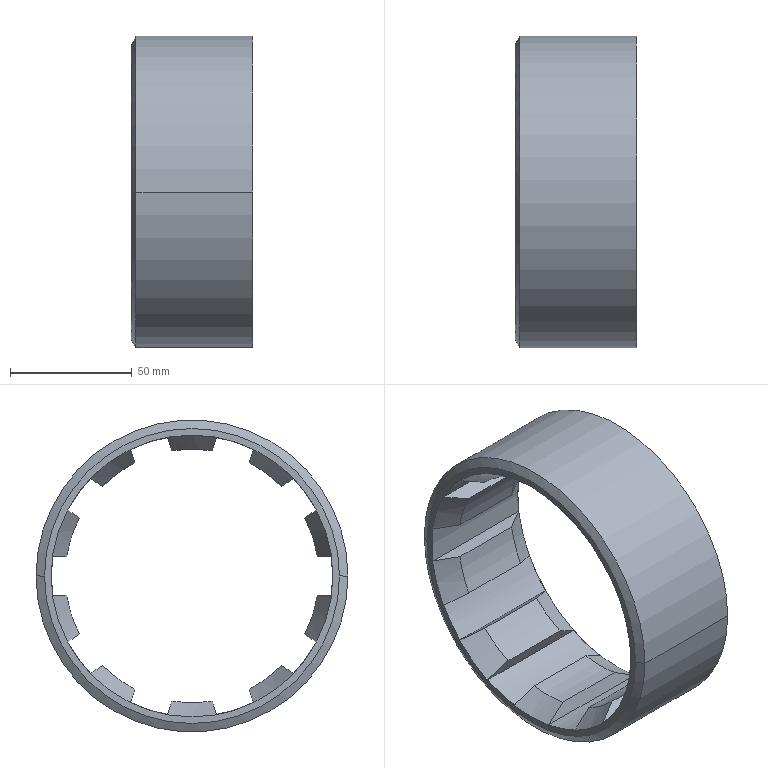Component | SolidWorks | RetainingRingSeatCenteringRing-1 | 1 solid | 50 faces | volume 161355 mm3 | cylinder 22 | plane 22 | cone 6 | commonest cylinder face diameters 104 x10 117 x10 128 x2 | material Alloy Steel